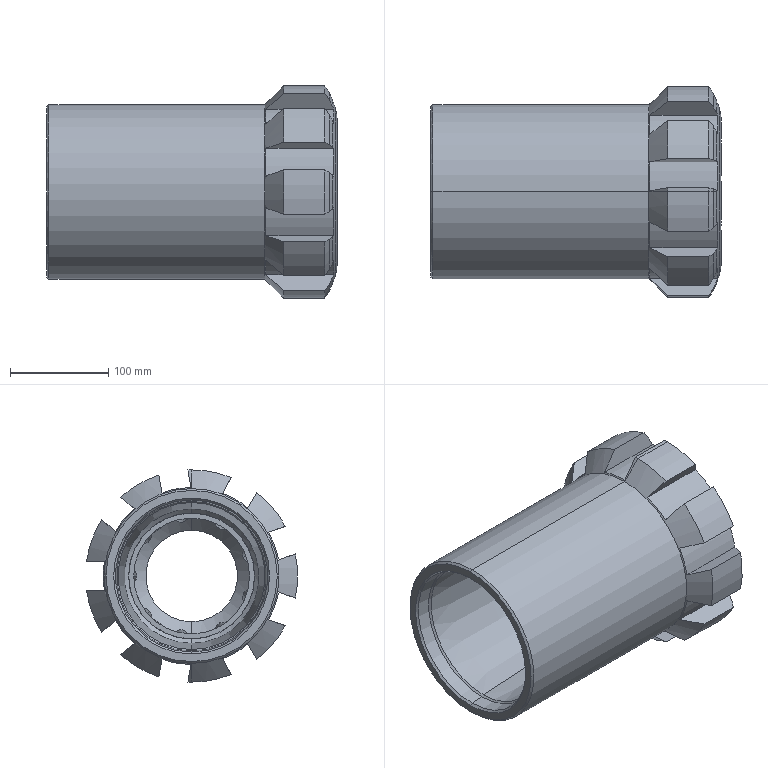Component | SolidWorks | DrillBit-1 | 1 solid | 135 faces | volume 3799005 mm3 | cone 58 | cylinder 47 | plane 30 | commonest cylinder face diameters 16 x18 215.983 x10 180 x9 128.01 x2 178 x2 93.423 x2 118 x2 128 x2 | material Alloy Steel